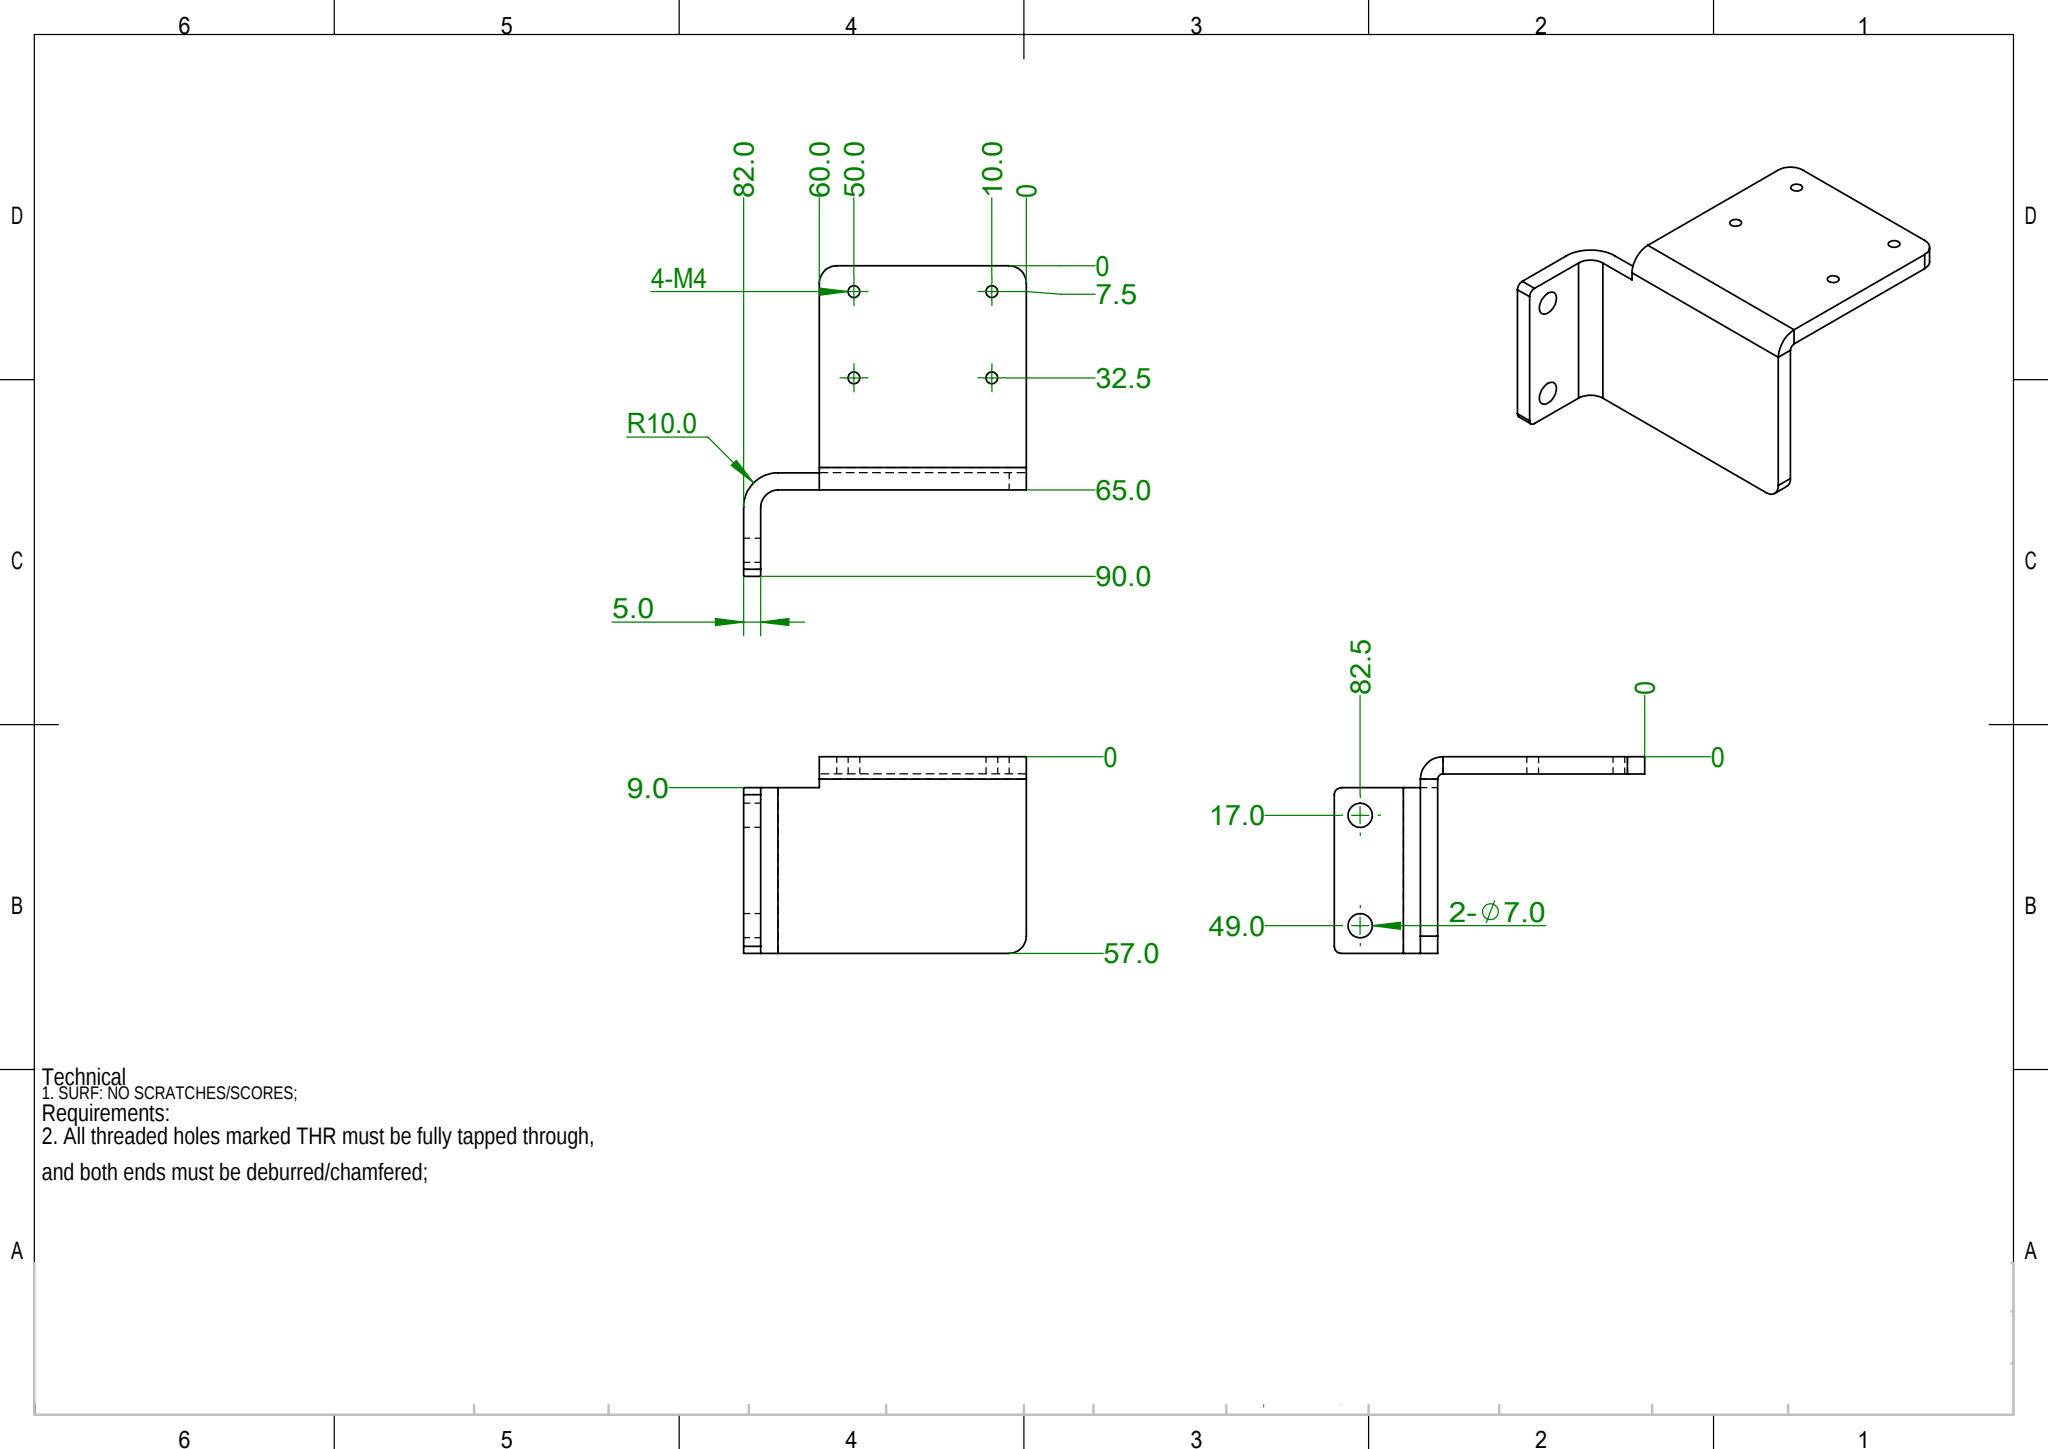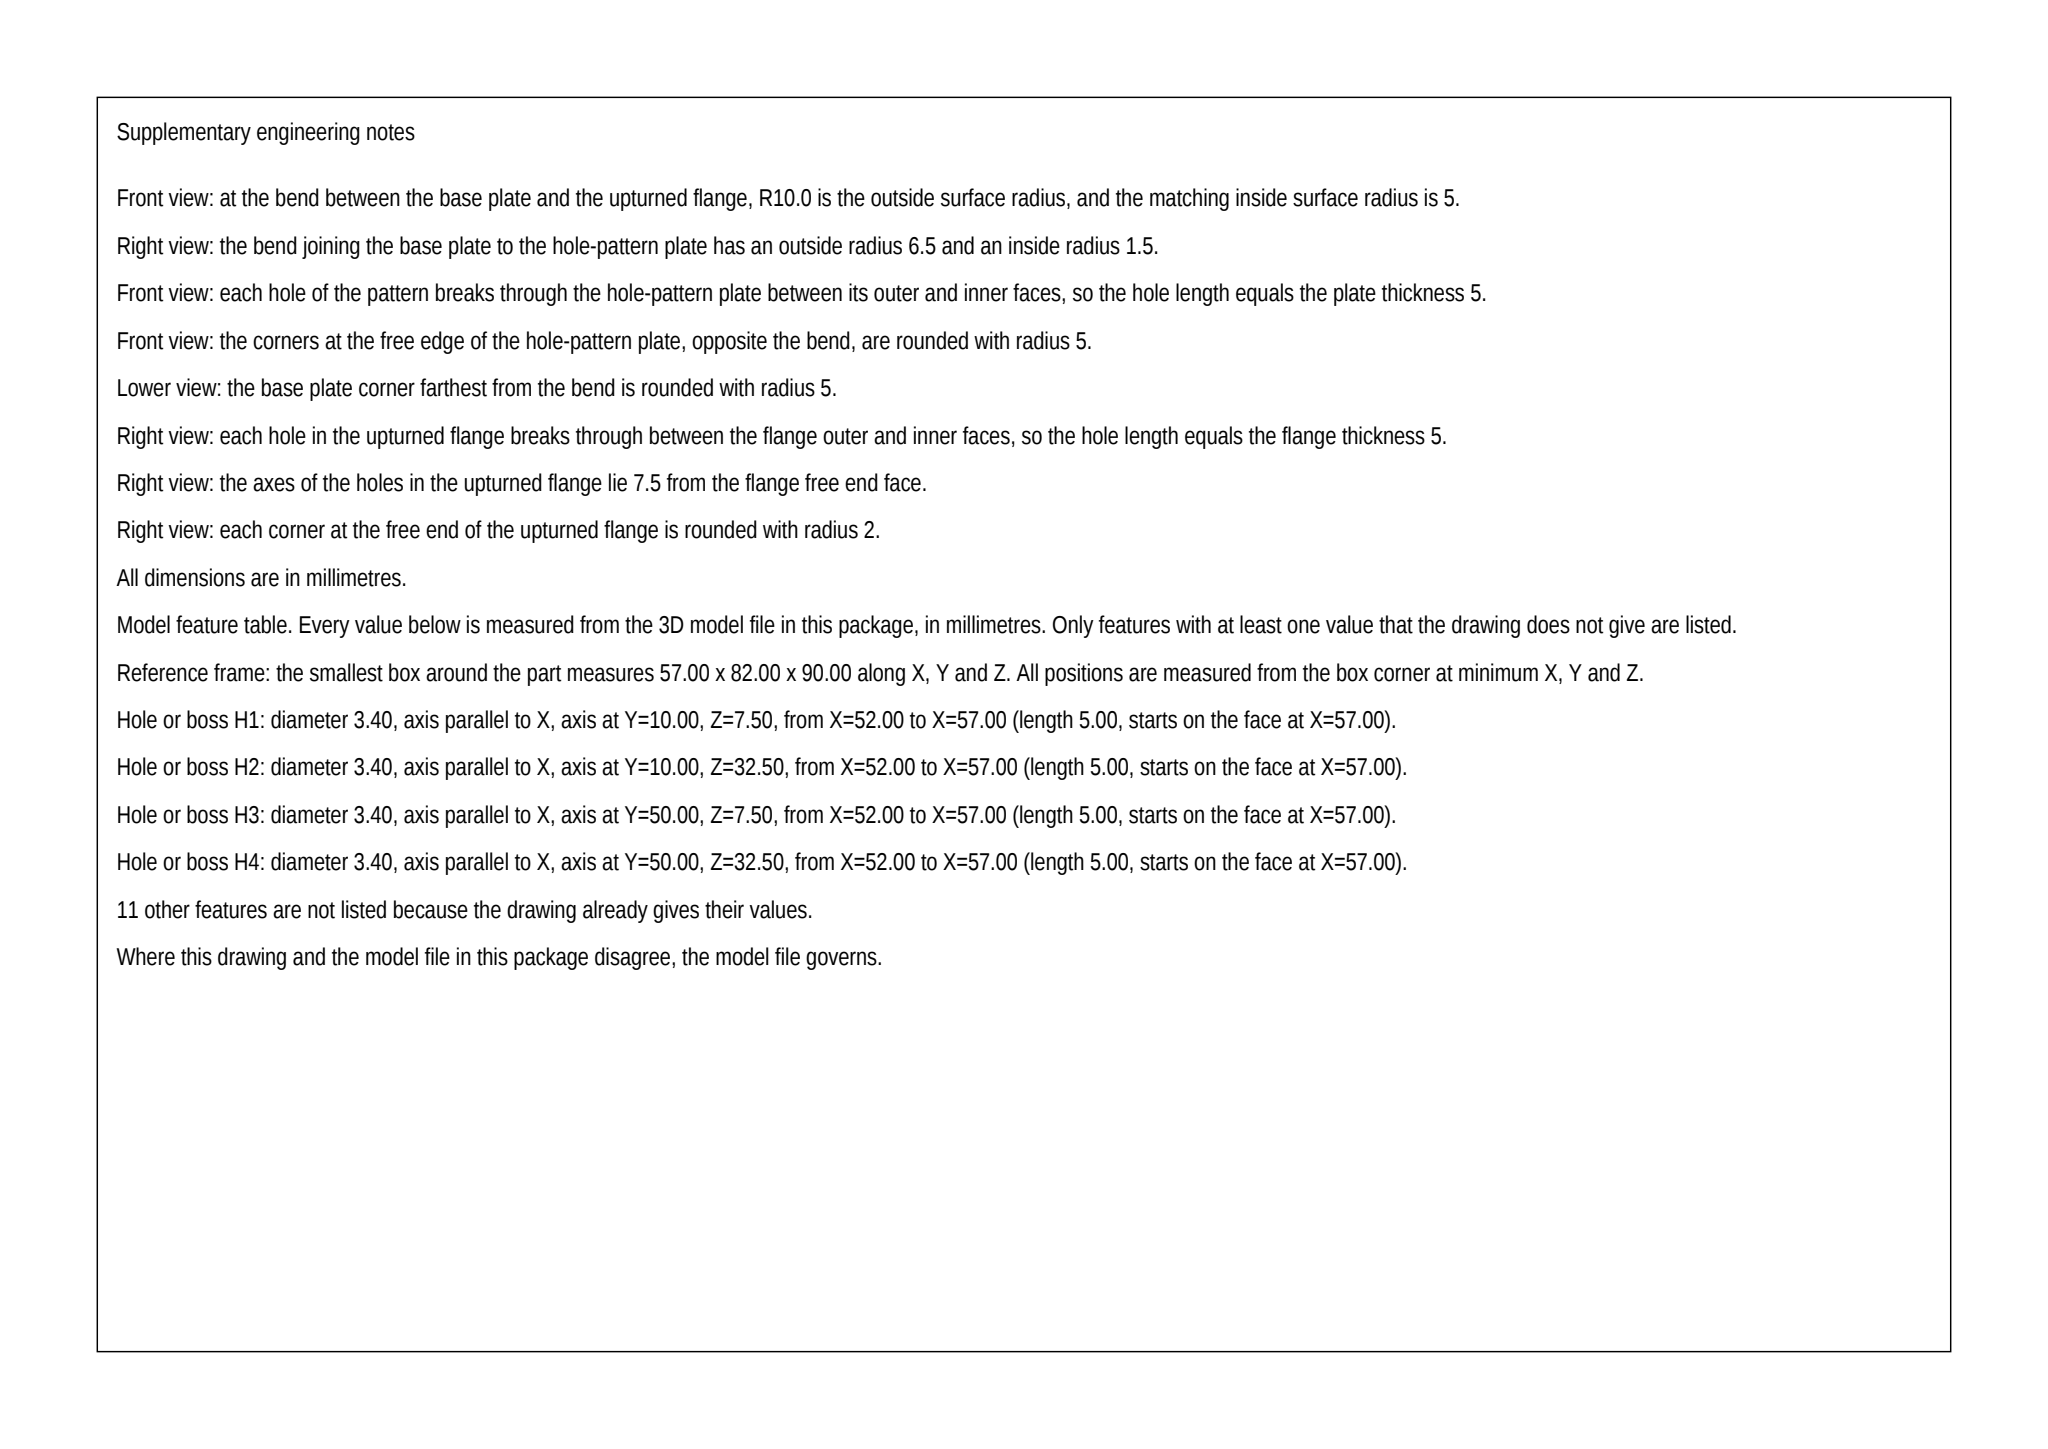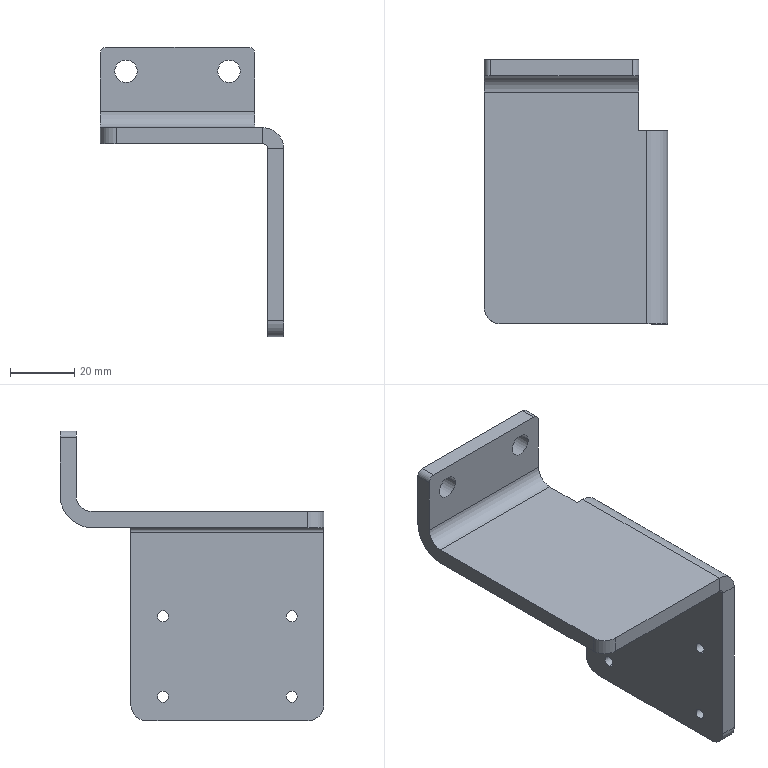Part | SolidWorks | mm | 1 solid | 37 faces | box 57 x 82 x 90 mm | volume 44437 mm3 | cylinder 21 | plane 16 | commonest cylinder face diameters 3.4 x8 7 x4 10 x4 4 x2 13 x1 3 x1 20 x1